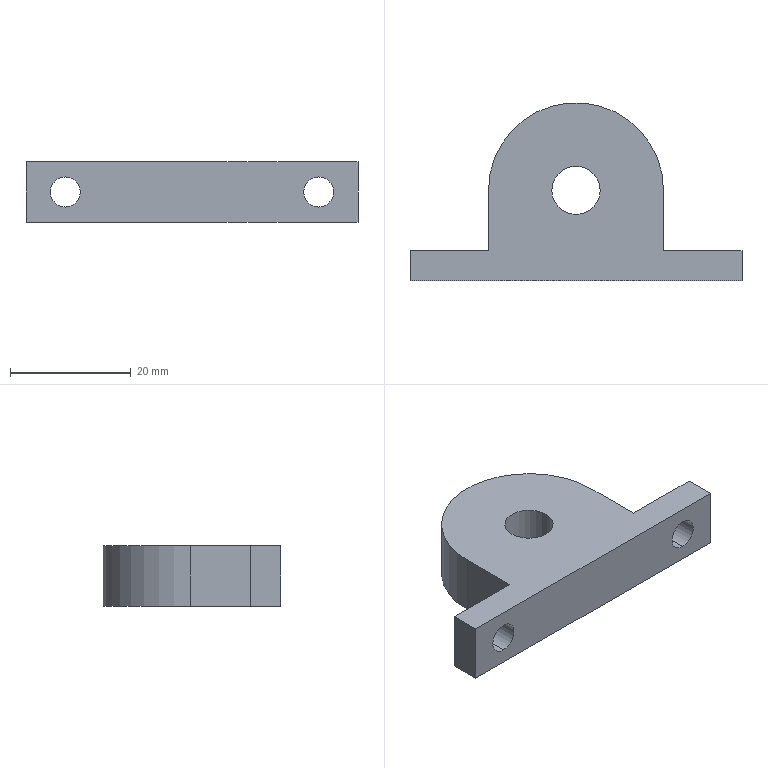Component | SolidWorks | BearingHousing-1 | 1 solid | 16 faces | box 55 x 29.5 x 10 mm | volume 8254 mm3 | plane 9 | cylinder 7 | commonest cylinder face diameters 5 x4 8 x2 29 x1
STEP:
#1=COLOUR_RGB('',0.7922,0.8196,0.9333);
#2=FILL_AREA_STYLE_COLOUR('',#1);
#3=FILL_AREA_STYLE('',(#2));
#4=SURFACE_STYLE_FILL_AREA(#3);
#5=SURFACE_SIDE_STYLE('',(#4));
#6=SURFACE_STYLE_USAGE(.BOTH.,#5);
#7=PRESENTATION_STYLE_ASSIGNMENT((#6));
#8=CARTESIAN_POINT('',(0.1575,0.,2.224));
#9=VERTEX_POINT('',#8);
#10=CARTESIAN_POINT('',(-0.1575,0.,2.224));
#11=VERTEX_POINT('',#10);
#12=CARTESIAN_POINT('',(0.,0.,2.224));
#13=DIRECTION('',(0.,0.,-1.));
#14=DIRECTION('',(-1.,0.,0.));
#15=AXIS2_PLACEMENT_3D('',#12,#13,#14);
#16=CIRCLE('',#15,0.1575);
#17=EDGE_CURVE('',#9,#11,#16,.T.);
#18=ORIENTED_EDGE('',*,*,#17,.F.);
#19=CARTESIAN_POINT('',(0.1575,0.,1.831));
#20=VERTEX_POINT('',#19);
#21=CARTESIAN_POINT('',(0.1575,0.,2.224));
#22=DIRECTION('',(0.,0.,-1.));
#23=VECTOR('',#22,39.37);
#24=LINE('',#21,#23);
#25=EDGE_CURVE('',#9,#20,#24,.T.);
#26=ORIENTED_EDGE('',*,*,#25,.T.);
#27=CARTESIAN_POINT('',(-0.1575,0.,1.831));
#28=VERTEX_POINT('',#27);
#29=CARTESIAN_POINT('',(0.,0.,1.831));
#30=DIRECTION('',(0.,0.,1.));
#31=DIRECTION('',(-1.,0.,0.));
#32=AXIS2_PLACEMENT_3D('',#29,#30,#31);
#33=CIRCLE('',#32,0.1575);
#34=EDGE_CURVE('',#28,#20,#33,.T.);
#35=ORIENTED_EDGE('',*,*,#34,.F.);
#36=CARTESIAN_POINT('',(-0.1575,0.,2.224));
#37=DIRECTION('',(0.,0.,-1.));
#38=VECTOR('',#37,39.37);
#39=LINE('',#36,#38);
#40=EDGE_CURVE('',#11,#28,#39,.T.);
#41=ORIENTED_EDGE('',*,*,#40,.F.);
#42=EDGE_LOOP('',(#18,#26,#35,#41));
#43=FACE_OUTER_BOUND('',#42,.T.);
#44=CARTESIAN_POINT('',(0.,0.,2.224));
#45=DIRECTION('',(0.,0.,-1.));
#46=DIRECTION('',(-1.,0.,0.));
#47=AXIS2_PLACEMENT_3D('',#44,#45,#46);
#48=CYLINDRICAL_SURFACE('',#47,0.1575);
#49=ADVANCED_FACE('',(#43),#48,.F.);
#50=CARTESIAN_POINT('',(-0.8268,-0.5906,2.126));
#51=VERTEX_POINT('',#50);
#52=CARTESIAN_POINT('',(-0.8268,-0.5906,1.929));
#53=VERTEX_POINT('',#52);
#54=CARTESIAN_POINT('',(-0.8268,-0.5906,2.028));
#55=DIRECTION('',(0.,-1.,0.));
#56=DIRECTION('',(0.,0.,1.));
#57=AXIS2_PLACEMENT_3D('',#54,#55,#56);
#58=CIRCLE('',#57,0.09843);
#59=EDGE_CURVE('',#51,#53,#58,.T.);
#60=ORIENTED_EDGE('',*,*,#59,.T.);
#61=CARTESIAN_POINT('',(-0.8268,-0.3937,1.929));
#62=VERTEX_POINT('',#61);
#63=CARTESIAN_POINT('',(-0.8268,-0.3937,1.929));
#64=DIRECTION('',(0.,1.,0.));
#65=VECTOR('',#64,39.37);
#66=LINE('',#63,#65);
#67=EDGE_CURVE('',#53,#62,#66,.T.);
#68=ORIENTED_EDGE('',*,*,#67,.T.);
#69=CARTESIAN_POINT('',(-0.8268,-0.3937,2.126));
#70=VERTEX_POINT('',#69);
#71=CARTESIAN_POINT('',(-0.8268,-0.3937,2.028));
#72=DIRECTION('',(0.,1.,0.));
#73=DIRECTION('',(0.,0.,1.));
#74=AXIS2_PLACEMENT_3D('',#71,#72,#73);
#75=CIRCLE('',#74,0.09843);
#76=EDGE_CURVE('',#62,#70,#75,.T.);
#77=ORIENTED_EDGE('',*,*,#76,.T.);
#78=CARTESIAN_POINT('',(-0.8268,-0.3937,2.126));
#79=DIRECTION('',(0.,1.,0.));
#80=VECTOR('',#79,39.37);
#81=LINE('',#78,#80);
#82=EDGE_CURVE('',#51,#70,#81,.T.);
#83=ORIENTED_EDGE('',*,*,#82,.F.);
#84=EDGE_LOOP('',(#60,#68,#77,#83));
#85=FACE_OUTER_BOUND('',#84,.T.);
#86=CARTESIAN_POINT('',(-0.8268,-0.3937,2.028));
#87=DIRECTION('',(0.,1.,0.));
#88=DIRECTION('',(0.,0.,1.));
#89=AXIS2_PLACEMENT_3D('',#86,#87,#88);
#90=CYLINDRICAL_SURFACE('',#89,0.09843);
#91=ADVANCED_FACE('',(#85),#90,.F.);
#92=CARTESIAN_POINT('',(0.8268,-0.5906,2.126));
#93=VERTEX_POINT('',#92);
#94=CARTESIAN_POINT('',(0.8268,-0.5906,1.929));
#95=VERTEX_POINT('',#94);
#96=CARTESIAN_POINT('',(0.8268,-0.5906,2.028));
#97=DIRECTION('',(0.,-1.,0.));
#98=DIRECTION('',(0.,0.,1.));
#99=AXIS2_PLACEMENT_3D('',#96,#97,#98);
#100=CIRCLE('',#99,0.09843);
#101=EDGE_CURVE('',#93,#95,#100,.T.);
#102=ORIENTED_EDGE('',*,*,#101,.T.);
#103=CARTESIAN_POINT('',(0.8268,-0.3937,1.929));
#104=VERTEX_POINT('',#103);
#105=CARTESIAN_POINT('',(0.8268,-0.3937,1.929));
#106=DIRECTION('',(0.,1.,0.));
#107=VECTOR('',#106,39.37);
#108=LINE('',#105,#107);
#109=EDGE_CURVE('',#95,#104,#108,.T.);
#110=ORIENTED_EDGE('',*,*,#109,.T.);
#111=CARTESIAN_POINT('',(0.8268,-0.3937,2.126));
#112=VERTEX_POINT('',#111);
#113=CARTESIAN_POINT('',(0.8268,-0.3937,2.028));
#114=DIRECTION('',(0.,1.,0.));
#115=DIRECTION('',(0.,0.,1.));
#116=AXIS2_PLACEMENT_3D('',#113,#114,#115);
#117=CIRCLE('',#116,0.09843);
#118=EDGE_CURVE('',#104,#112,#117,.T.);
#119=ORIENTED_EDGE('',*,*,#118,.T.);
#120=CARTESIAN_POINT('',(0.8268,-0.3937,2.126));
#121=DIRECTION('',(0.,1.,0.));
#122=VECTOR('',#121,39.37);
#123=LINE('',#120,#122);
#124=EDGE_CURVE('',#93,#112,#123,.T.);
#125=ORIENTED_EDGE('',*,*,#124,.F.);
#126=EDGE_LOOP('',(#102,#110,#119,#125));
#127=FACE_OUTER_BOUND('',#126,.T.);
#128=CARTESIAN_POINT('',(0.8268,-0.3937,2.028));
#129=DIRECTION('',(0.,1.,0.));
#130=DIRECTION('',(0.,0.,1.));
#131=AXIS2_PLACEMENT_3D('',#128,#129,#130);
#132=CYLINDRICAL_SURFACE('',#131,0.09843);
#133=ADVANCED_FACE('',(#127),#132,.F.);
#134=CARTESIAN_POINT('',(0.,0.,2.224));
#135=DIRECTION('',(0.,0.,-1.));
#136=DIRECTION('',(-1.,0.,0.));
#137=AXIS2_PLACEMENT_3D('',#134,#135,#136);
#138=CIRCLE('',#137,0.1575);
#139=EDGE_CURVE('',#11,#9,#138,.T.);
#140=ORIENTED_EDGE('',*,*,#139,.T.);
#141=ORIENTED_EDGE('',*,*,#17,.T.);
#142=EDGE_LOOP('',(#140,#141));
#143=FACE_BOUND('',#142,.T.);
#144=CARTESIAN_POINT('',(-0.5709,-0.3937,2.224));
#145=VERTEX_POINT('',#144);
#146=CARTESIAN_POINT('',(-1.083,-0.3937,2.224));
#147=VERTEX_POINT('',#146);
#148=CARTESIAN_POINT('',(0.,-0.3937,2.224));
#149=DIRECTION('',(-1.,0.,0.));
#150=VECTOR('',#149,39.37);
#151=LINE('',#148,#150);
#152=EDGE_CURVE('',#145,#147,#151,.T.);
#153=ORIENTED_EDGE('',*,*,#152,.T.);
#154=CARTESIAN_POINT('',(-1.083,-0.5906,2.224));
#155=VERTEX_POINT('',#154);
#156=CARTESIAN_POINT('',(-1.083,0.,2.224));
#157=DIRECTION('',(0.,-1.,0.));
#158=VECTOR('',#157,39.37);
#159=LINE('',#156,#158);
#160=EDGE_CURVE('',#147,#155,#159,.T.);
#161=ORIENTED_EDGE('',*,*,#160,.T.);
#162=CARTESIAN_POINT('',(1.083,-0.5906,2.224));
#163=VERTEX_POINT('',#162);
#164=CARTESIAN_POINT('',(0.,-0.5906,2.224));
#165=DIRECTION('',(1.,0.,0.));
#166=VECTOR('',#165,39.37);
#167=LINE('',#164,#166);
#168=EDGE_CURVE('',#155,#163,#167,.T.);
#169=ORIENTED_EDGE('',*,*,#168,.T.);
#170=CARTESIAN_POINT('',(1.083,-0.3937,2.224));
#171=VERTEX_POINT('',#170);
#172=CARTESIAN_POINT('',(1.083,0.,2.224));
#173=DIRECTION('',(0.,1.,0.));
#174=VECTOR('',#173,39.37);
#175=LINE('',#172,#174);
#176=EDGE_CURVE('',#163,#171,#175,.T.);
#177=ORIENTED_EDGE('',*,*,#176,.T.);
#178=CARTESIAN_POINT('',(0.5709,-0.3937,2.224));
#179=VERTEX_POINT('',#178);
#180=CARTESIAN_POINT('',(0.,-0.3937,2.224));
#181=DIRECTION('',(-1.,0.,0.));
#182=VECTOR('',#181,39.37);
#183=LINE('',#180,#182);
#184=EDGE_CURVE('',#171,#179,#183,.T.);
#185=ORIENTED_EDGE('',*,*,#184,.T.);
#186=CARTESIAN_POINT('',(0.5709,0.,2.224));
#187=VERTEX_POINT('',#186);
#188=CARTESIAN_POINT('',(0.5709,0.,2.224));
#189=DIRECTION('',(0.,1.,0.));
#190=VECTOR('',#189,39.37);
#191=LINE('',#188,#190);
#192=EDGE_CURVE('',#179,#187,#191,.T.);
#193=ORIENTED_EDGE('',*,*,#192,.T.);
#194=CARTESIAN_POINT('',(-0.5709,0.,2.224));
#195=VERTEX_POINT('',#194);
#196=CARTESIAN_POINT('',(0.,0.,2.224));
#197=DIRECTION('',(0.,0.,1.));
#198=DIRECTION('',(-1.,0.,0.));
#199=AXIS2_PLACEMENT_3D('',#196,#197,#198);
#200=CIRCLE('',#199,0.5709);
#201=EDGE_CURVE('',#187,#195,#200,.T.);
#202=ORIENTED_EDGE('',*,*,#201,.T.);
#203=CARTESIAN_POINT('',(-0.5709,0.,2.224));
#204=DIRECTION('',(0.,-1.,0.));
#205=VECTOR('',#204,39.37);
#206=LINE('',#203,#205);
#207=EDGE_CURVE('',#195,#145,#206,.T.);
#208=ORIENTED_EDGE('',*,*,#207,.T.);
#209=EDGE_LOOP('',(#153,#161,#169,#177,#185,#193,#202,#208));
#210=FACE_OUTER_BOUND('',#209,.T.);
#211=CARTESIAN_POINT('',(0.,0.,2.224));
#212=DIRECTION('',(0.,0.,1.));
#213=DIRECTION('',(1.,0.,0.));
#214=AXIS2_PLACEMENT_3D('',#211,#212,#213);
#215=PLANE('',#214);
#216=ADVANCED_FACE('',(#143,#210),#215,.T.);
#217=ORIENTED_EDGE('',*,*,#25,.F.);
#218=ORIENTED_EDGE('',*,*,#139,.F.);
#219=ORIENTED_EDGE('',*,*,#40,.T.);
#220=CARTESIAN_POINT('',(0.,0.,1.831));
#221=DIRECTION('',(0.,0.,1.));
#222=DIRECTION('',(-1.,0.,0.));
#223=AXIS2_PLACEMENT_3D('',#220,#221,#222);
#224=CIRCLE('',#223,0.1575);
#225=EDGE_CURVE('',#20,#28,#224,.T.);
#226=ORIENTED_EDGE('',*,*,#225,.F.);
#227=EDGE_LOOP('',(#217,#218,#219,#226));
#228=FACE_OUTER_BOUND('',#227,.T.);
#229=CARTESIAN_POINT('',(0.,0.,2.224));
#230=DIRECTION('',(0.,0.,-1.));
#231=DIRECTION('',(-1.,0.,0.));
#232=AXIS2_PLACEMENT_3D('',#229,#230,#231);
#233=CYLINDRICAL_SURFACE('',#232,0.1575);
#234=ADVANCED_FACE('',(#228),#233,.F.);
#235=CARTESIAN_POINT('',(-1.083,-0.5906,1.831));
#236=VERTEX_POINT('',#235);
#237=CARTESIAN_POINT('',(-1.083,-0.5906,2.224));
#238=DIRECTION('',(0.,0.,-1.));
#239=VECTOR('',#238,39.37);
#240=LINE('',#237,#239);
#241=EDGE_CURVE('',#155,#236,#240,.T.);
#242=ORIENTED_EDGE('',*,*,#241,.F.);
#243=ORIENTED_EDGE('',*,*,#160,.F.);
#244=CARTESIAN_POINT('',(-1.083,-0.3937,1.831));
#245=VERTEX_POINT('',#244);
#246=CARTESIAN_POINT('',(-1.083,-0.3937,2.224));
#247=DIRECTION('',(0.,0.,1.));
#248=VECTOR('',#247,39.37);
#249=LINE('',#246,#248);
#250=EDGE_CURVE('',#245,#147,#249,.T.);
#251=ORIENTED_EDGE('',*,*,#250,.F.);
#252=CARTESIAN_POINT('',(-1.083,-0.3937,1.831));
#253=DIRECTION('',(0.,1.,0.));
#254=VECTOR('',#253,39.37);
#255=LINE('',#252,#254);
#256=EDGE_CURVE('',#236,#245,#255,.T.);
#257=ORIENTED_EDGE('',*,*,#256,.F.);
#258=EDGE_LOOP('',(#242,#243,#251,#257));
#259=FACE_OUTER_BOUND('',#258,.T.);
#260=CARTESIAN_POINT('',(-1.083,-0.3937,2.224));
#261=DIRECTION('',(1.,0.,0.));
#262=DIRECTION('',(0.,0.,-1.));
#263=AXIS2_PLACEMENT_3D('',#260,#261,#262);
#264=PLANE('',#263);
#265=ADVANCED_FACE('',(#259),#264,.F.);
#266=ORIENTED_EDGE('',*,*,#250,.T.);
#267=ORIENTED_EDGE('',*,*,#152,.F.);
#268=CARTESIAN_POINT('',(-0.5709,-0.3937,1.831));
#269=VERTEX_POINT('',#268);
#270=CARTESIAN_POINT('',(-0.5709,-0.3937,2.224));
#271=DIRECTION('',(0.,0.,1.));
#272=VECTOR('',#271,39.37);
#273=LINE('',#270,#272);
#274=EDGE_CURVE('',#269,#145,#273,.T.);
#275=ORIENTED_EDGE('',*,*,#274,.F.);
#276=CARTESIAN_POINT('',(-0.5709,-0.3937,1.831));
#277=DIRECTION('',(1.,-0.,0.));
#278=VECTOR('',#277,39.37);
#279=LINE('',#276,#278);
#280=EDGE_CURVE('',#245,#269,#279,.T.);
#281=ORIENTED_EDGE('',*,*,#280,.F.);
#282=EDGE_LOOP('',(#266,#267,#275,#281));
#283=FACE_OUTER_BOUND('',#282,.T.);
#284=CARTESIAN_POINT('',(-0.8268,-0.3937,2.028));
#285=DIRECTION('',(0.,1.,0.));
#286=DIRECTION('',(0.,0.,1.));
#287=AXIS2_PLACEMENT_3D('',#284,#285,#286);
#288=CIRCLE('',#287,0.09843);
#289=EDGE_CURVE('',#70,#62,#288,.T.);
#290=ORIENTED_EDGE('',*,*,#289,.F.);
#291=ORIENTED_EDGE('',*,*,#76,.F.);
#292=EDGE_LOOP('',(#290,#291));
#293=FACE_BOUND('',#292,.T.);
#294=CARTESIAN_POINT('',(-0.5709,-0.3937,2.224));
#295=DIRECTION('',(-0.,-1.,0.));
#296=DIRECTION('',(1.,-0.,0.));
#297=AXIS2_PLACEMENT_3D('',#294,#295,#296);
#298=PLANE('',#297);
#299=ADVANCED_FACE('',(#283,#293),#298,.F.);
#300=ORIENTED_EDGE('',*,*,#274,.T.);
#301=ORIENTED_EDGE('',*,*,#207,.F.);
#302=CARTESIAN_POINT('',(-0.5709,0.,1.831));
#303=VERTEX_POINT('',#302);
#304=CARTESIAN_POINT('',(-0.5709,0.,2.224));
#305=DIRECTION('',(0.,0.,1.));
#306=VECTOR('',#305,39.37);
#307=LINE('',#304,#306);
#308=EDGE_CURVE('',#303,#195,#307,.T.);
#309=ORIENTED_EDGE('',*,*,#308,.F.);
#310=CARTESIAN_POINT('',(-0.5709,0.,1.831));
#311=DIRECTION('',(-0.,1.,0.));
#312=VECTOR('',#311,39.37);
#313=LINE('',#310,#312);
#314=EDGE_CURVE('',#269,#303,#313,.T.);
#315=ORIENTED_EDGE('',*,*,#314,.F.);
#316=EDGE_LOOP('',(#300,#301,#309,#315));
#317=FACE_OUTER_BOUND('',#316,.T.);
#318=CARTESIAN_POINT('',(-0.5709,0.,2.224));
#319=DIRECTION('',(1.,0.,0.));
#320=DIRECTION('',(-0.,1.,0.));
#321=AXIS2_PLACEMENT_3D('',#318,#319,#320);
#322=PLANE('',#321);
#323=ADVANCED_FACE('',(#317),#322,.F.);
#324=ORIENTED_EDGE('',*,*,#201,.F.);
#325=CARTESIAN_POINT('',(0.5709,-0.,1.831));
#326=VERTEX_POINT('',#325);
#327=CARTESIAN_POINT('',(0.5709,0.,2.224));
#328=DIRECTION('',(0.,0.,-1.));
#329=VECTOR('',#328,39.37);
#330=LINE('',#327,#329);
#331=EDGE_CURVE('',#187,#326,#330,.T.);
#332=ORIENTED_EDGE('',*,*,#331,.T.);
#333=CARTESIAN_POINT('',(0.,0.,1.831));
#334=DIRECTION('',(0.,0.,1.));
#335=DIRECTION('',(-1.,0.,0.));
#336=AXIS2_PLACEMENT_3D('',#333,#334,#335);
#337=CIRCLE('',#336,0.5709);
#338=EDGE_CURVE('',#326,#303,#337,.T.);
#339=ORIENTED_EDGE('',*,*,#338,.T.);
#340=ORIENTED_EDGE('',*,*,#308,.T.);
#341=EDGE_LOOP('',(#324,#332,#339,#340));
#342=FACE_OUTER_BOUND('',#341,.T.);
#343=CARTESIAN_POINT('',(0.,0.,2.224));
#344=DIRECTION('',(0.,0.,-1.));
#345=DIRECTION('',(-1.,0.,0.));
#346=AXIS2_PLACEMENT_3D('',#343,#344,#345);
#347=CYLINDRICAL_SURFACE('',#346,0.5709);
#348=ADVANCED_FACE('',(#342),#347,.T.);
#349=ORIENTED_EDGE('',*,*,#331,.F.);
#350=ORIENTED_EDGE('',*,*,#192,.F.);
#351=CARTESIAN_POINT('',(0.5709,-0.3937,1.831));
#352=VERTEX_POINT('',#351);
#353=CARTESIAN_POINT('',(0.5709,-0.3937,2.224));
#354=DIRECTION('',(0.,0.,1.));
#355=VECTOR('',#354,39.37);
#356=LINE('',#353,#355);
#357=EDGE_CURVE('',#352,#179,#356,.T.);
#358=ORIENTED_EDGE('',*,*,#357,.F.);
#359=CARTESIAN_POINT('',(0.5709,0.,1.831));
#360=DIRECTION('',(-0.,-1.,0.));
#361=VECTOR('',#360,39.37);
#362=LINE('',#359,#361);
#363=EDGE_CURVE('',#326,#352,#362,.T.);
#364=ORIENTED_EDGE('',*,*,#363,.F.);
#365=EDGE_LOOP('',(#349,#350,#358,#364));
#366=FACE_OUTER_BOUND('',#365,.T.);
#367=CARTESIAN_POINT('',(0.5709,0.,2.224));
#368=DIRECTION('',(-1.,0.,0.));
#369=DIRECTION('',(-0.,-1.,0.));
#370=AXIS2_PLACEMENT_3D('',#367,#368,#369);
#371=PLANE('',#370);
#372=ADVANCED_FACE('',(#366),#371,.F.);
#373=ORIENTED_EDGE('',*,*,#357,.T.);
#374=ORIENTED_EDGE('',*,*,#184,.F.);
#375=CARTESIAN_POINT('',(1.083,-0.3937,1.831));
#376=VERTEX_POINT('',#375);
#377=CARTESIAN_POINT('',(1.083,-0.3937,2.224));
#378=DIRECTION('',(0.,0.,1.));
#379=VECTOR('',#378,39.37);
#380=LINE('',#377,#379);
#381=EDGE_CURVE('',#376,#171,#380,.T.);
#382=ORIENTED_EDGE('',*,*,#381,.F.);
#383=CARTESIAN_POINT('',(0.5709,-0.3937,1.831));
#384=DIRECTION('',(1.,0.,0.));
#385=VECTOR('',#384,39.37);
#386=LINE('',#383,#385);
#387=EDGE_CURVE('',#352,#376,#386,.T.);
#388=ORIENTED_EDGE('',*,*,#387,.F.);
#389=EDGE_LOOP('',(#373,#374,#382,#388));
#390=FACE_OUTER_BOUND('',#389,.T.);
#391=CARTESIAN_POINT('',(0.8268,-0.3937,2.028));
#392=DIRECTION('',(0.,1.,0.));
#393=DIRECTION('',(0.,0.,1.));
#394=AXIS2_PLACEMENT_3D('',#391,#392,#393);
#395=CIRCLE('',#394,0.09843);
#396=EDGE_CURVE('',#112,#104,#395,.T.);
#397=ORIENTED_EDGE('',*,*,#396,.F.);
#398=ORIENTED_EDGE('',*,*,#118,.F.);
#399=EDGE_LOOP('',(#397,#398));
#400=FACE_BOUND('',#399,.T.);
#401=CARTESIAN_POINT('',(0.5709,-0.3937,2.224));
#402=DIRECTION('',(0.,-1.,0.));
#403=DIRECTION('',(1.,0.,0.));
#404=AXIS2_PLACEMENT_3D('',#401,#402,#403);
#405=PLANE('',#404);
#406=ADVANCED_FACE('',(#390,#400),#405,.F.);
#407=ORIENTED_EDGE('',*,*,#381,.T.);
#408=ORIENTED_EDGE('',*,*,#176,.F.);
#409=CARTESIAN_POINT('',(1.083,-0.5906,1.831));
#410=VERTEX_POINT('',#409);
#411=CARTESIAN_POINT('',(1.083,-0.5906,2.224));
#412=DIRECTION('',(0.,0.,1.));
#413=VECTOR('',#412,39.37);
#414=LINE('',#411,#413);
#415=EDGE_CURVE('',#410,#163,#414,.T.);
#416=ORIENTED_EDGE('',*,*,#415,.F.);
#417=CARTESIAN_POINT('',(1.083,-0.3937,1.831));
#418=DIRECTION('',(0.,-1.,0.));
#419=VECTOR('',#418,39.37);
#420=LINE('',#417,#419);
#421=EDGE_CURVE('',#376,#410,#420,.T.);
#422=ORIENTED_EDGE('',*,*,#421,.F.);
#423=EDGE_LOOP('',(#407,#408,#416,#422));
#424=FACE_OUTER_BOUND('',#423,.T.);
#425=CARTESIAN_POINT('',(1.083,-0.3937,2.224));
#426=DIRECTION('',(-1.,0.,0.));
#427=DIRECTION('',(0.,0.,1.));
#428=AXIS2_PLACEMENT_3D('',#425,#426,#427);
#429=PLANE('',#428);
#430=ADVANCED_FACE('',(#424),#429,.F.);
#431=ORIENTED_EDGE('',*,*,#415,.T.);
#432=ORIENTED_EDGE('',*,*,#168,.F.);
#433=ORIENTED_EDGE('',*,*,#241,.T.);
#434=CARTESIAN_POINT('',(-1.083,-0.5906,1.831));
#435=DIRECTION('',(-1.,0.,0.));
#436=VECTOR('',#435,39.37);
#437=LINE('',#434,#436);
#438=EDGE_CURVE('',#410,#236,#437,.T.);
#439=ORIENTED_EDGE('',*,*,#438,.F.);
#440=EDGE_LOOP('',(#431,#432,#433,#439));
#441=FACE_OUTER_BOUND('',#440,.T.);
#442=ORIENTED_EDGE('',*,*,#59,.F.);
#443=CARTESIAN_POINT('',(-0.8268,-0.5906,2.028));
#444=DIRECTION('',(0.,-1.,0.));
#445=DIRECTION('',(0.,0.,1.));
#446=AXIS2_PLACEMENT_3D('',#443,#444,#445);
#447=CIRCLE('',#446,0.09843);
#448=EDGE_CURVE('',#53,#51,#447,.T.);
#449=ORIENTED_EDGE('',*,*,#448,.F.);
#450=EDGE_LOOP('',(#442,#449));
#451=FACE_BOUND('',#450,.T.);
#452=ORIENTED_EDGE('',*,*,#101,.F.);
#453=CARTESIAN_POINT('',(0.8268,-0.5906,2.028));
#454=DIRECTION('',(0.,-1.,0.));
#455=DIRECTION('',(0.,0.,1.));
#456=AXIS2_PLACEMENT_3D('',#453,#454,#455);
#457=CIRCLE('',#456,0.09843);
#458=EDGE_CURVE('',#95,#93,#457,.T.);
#459=ORIENTED_EDGE('',*,*,#458,.F.);
#460=EDGE_LOOP('',(#452,#459));
#461=FACE_BOUND('',#460,.T.);
#462=CARTESIAN_POINT('',(-1.083,-0.5906,2.224));
#463=DIRECTION('',(0.,1.,0.));
#464=DIRECTION('',(0.,0.,1.));
#465=AXIS2_PLACEMENT_3D('',#462,#463,#464);
#466=PLANE('',#465);
#467=ADVANCED_FACE('',(#441,#451,#461),#466,.F.);
#468=ORIENTED_EDGE('',*,*,#34,.T.);
#469=ORIENTED_EDGE('',*,*,#225,.T.);
#470=EDGE_LOOP('',(#468,#469));
#471=FACE_BOUND('',#470,.T.);
#472=ORIENTED_EDGE('',*,*,#256,.T.);
#473=ORIENTED_EDGE('',*,*,#280,.T.);
#474=ORIENTED_EDGE('',*,*,#314,.T.);
#475=ORIENTED_EDGE('',*,*,#338,.F.);
#476=ORIENTED_EDGE('',*,*,#363,.T.);
#477=ORIENTED_EDGE('',*,*,#387,.T.);
#478=ORIENTED_EDGE('',*,*,#421,.T.);
#479=ORIENTED_EDGE('',*,*,#438,.T.);
#480=EDGE_LOOP('',(#472,#473,#474,#475,#476,#477,#478,#479));
#481=FACE_OUTER_BOUND('',#480,.T.);
#482=CARTESIAN_POINT('',(0.,0.,1.831));
#483=DIRECTION('',(0.,0.,1.));
#484=DIRECTION('',(1.,0.,0.));
#485=AXIS2_PLACEMENT_3D('',#482,#483,#484);
#486=PLANE('',#485);
#487=ADVANCED_FACE('',(#471,#481),#486,.F.);
#488=ORIENTED_EDGE('',*,*,#67,.F.);
#489=ORIENTED_EDGE('',*,*,#448,.T.);
#490=ORIENTED_EDGE('',*,*,#82,.T.);
#491=ORIENTED_EDGE('',*,*,#289,.T.);
#492=EDGE_LOOP('',(#488,#489,#490,#491));
#493=FACE_OUTER_BOUND('',#492,.T.);
#494=CARTESIAN_POINT('',(-0.8268,-0.3937,2.028));
#495=DIRECTION('',(0.,1.,0.));
#496=DIRECTION('',(0.,0.,1.));
#497=AXIS2_PLACEMENT_3D('',#494,#495,#496);
#498=CYLINDRICAL_SURFACE('',#497,0.09843);
#499=ADVANCED_FACE('',(#493),#498,.F.);
#500=ORIENTED_EDGE('',*,*,#109,.F.);
#501=ORIENTED_EDGE('',*,*,#458,.T.);
#502=ORIENTED_EDGE('',*,*,#124,.T.);
#503=ORIENTED_EDGE('',*,*,#396,.T.);
#504=EDGE_LOOP('',(#500,#501,#502,#503));
#505=FACE_OUTER_BOUND('',#504,.T.);
#506=CARTESIAN_POINT('',(0.8268,-0.3937,2.028));
#507=DIRECTION('',(0.,1.,0.));
#508=DIRECTION('',(0.,0.,1.));
#509=AXIS2_PLACEMENT_3D('',#506,#507,#508);
#510=CYLINDRICAL_SURFACE('',#509,0.09843);
#511=ADVANCED_FACE('',(#505),#510,.F.);
#512=CLOSED_SHELL('',(#49,#91,#133,#216,#234,#265,#299,#323,#348,#372,#406,#430,#467,#487,#499,#511));
#513=MANIFOLD_SOLID_BREP('',#512);
#514=STYLED_ITEM('',(#7),#513);
#515=(LENGTH_UNIT()NAMED_UNIT(*)SI_UNIT($,.METRE.));
#516=LENGTH_MEASURE_WITH_UNIT(LENGTH_MEASURE(0.0254),#515);
#517=DIMENSIONAL_EXPONENTS(1.,0.,0.,0.,0.,0.,0.);
#518=(CONVERSION_BASED_UNIT('',#516)LENGTH_UNIT()NAMED_UNIT(#517));
#519=UNCERTAINTY_MEASURE_WITH_UNIT(LENGTH_MEASURE(0.00001),#518,'','');
#520=(NAMED_UNIT(*)PLANE_ANGLE_UNIT()SI_UNIT($,.RADIAN.));
#521=(NAMED_UNIT(*)SI_UNIT($,.STERADIAN.)SOLID_ANGLE_UNIT());
#522=(GEOMETRIC_REPRESENTATION_CONTEXT(3)GLOBAL_UNCERTAINTY_ASSIGNED_CONTEXT((#519))GLOBAL_UNIT_ASSIGNED_CONTEXT((#518,#520,#521))REPRESENTATION_CONTEXT('',''));
#523=MECHANICAL_DESIGN_GEOMETRIC_PRESENTATION_REPRESENTATION('',(#514),#522);
#524=PRESENTATION_LAYER_ASSIGNMENT('','',(#514));
#525=CARTESIAN_POINT('',(0.,0.,0.));
#526=DIRECTION('',(0.,0.,1.));
#527=DIRECTION('',(1.,0.,0.));
#528=AXIS2_PLACEMENT_3D('',#525,#526,#527);
#529=(LENGTH_UNIT()NAMED_UNIT(*)SI_UNIT($,.METRE.));
#530=LENGTH_MEASURE_WITH_UNIT(LENGTH_MEASURE(0.0254),#529);
#531=DIMENSIONAL_EXPONENTS(1.,0.,0.,0.,0.,0.,0.);
#532=(CONVERSION_BASED_UNIT('',#530)LENGTH_UNIT()NAMED_UNIT(#531));
#533=UNCERTAINTY_MEASURE_WITH_UNIT(LENGTH_MEASURE(0.00001),#532,'','');
#534=(NAMED_UNIT(*)PLANE_ANGLE_UNIT()SI_UNIT($,.RADIAN.));
#535=(NAMED_UNIT(*)SI_UNIT($,.STERADIAN.)SOLID_ANGLE_UNIT());
#536=(GEOMETRIC_REPRESENTATION_CONTEXT(3)GLOBAL_UNCERTAINTY_ASSIGNED_CONTEXT((#533))GLOBAL_UNIT_ASSIGNED_CONTEXT((#532,#534,#535))REPRESENTATION_CONTEXT('',''));
#537=ADVANCED_BREP_SHAPE_REPRESENTATION('',(#513,#528),#536);